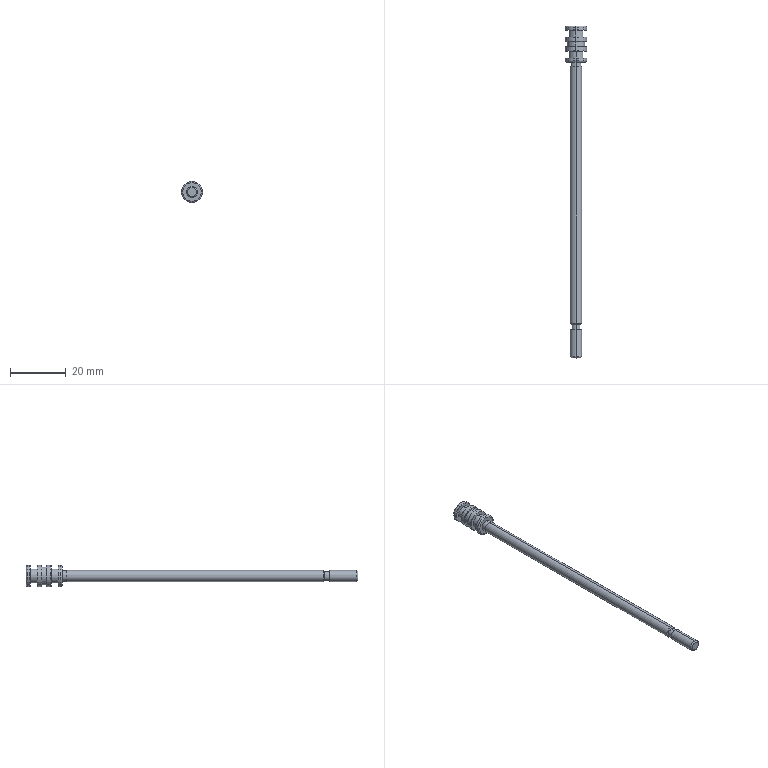Component | SolidWorks | MI-8x60-S-U-M-2(0)-1_MI 8x60-S-U_r-1 | 1 solid | 53 faces | box 7.6 x 119 x 7.6 mm | volume 1755 mm3 | cylinder 22 | cone 16 | plane 11 | torus 4 | commonest cylinder face diameters 7.6 x8 5 x4 4 x4 6.3 x2 3.9 x2 3.2 x2
build123d program:
from build123d import *


with BuildPart() as part:
    # Sketch1 → Revolve1 (revolve)
    with BuildSketch(Plane.XY, mode=Mode.PRIVATE) as revolve1_sk:
        with BuildLine():
            Line((-28, 0), (-28, 1.571))
            Line((-28, 1.571), (-27.57, 2))
            Line((-27.57, 2), (-17.8, 2))
            Line((-17.8, 2), (-17.8, 1.6))
            Line((-17.8, 1.6), (-16, 1.6))
            Line((-16, 1.6), (-15.6, 2))
            Line((-15.6, 2), (76.5, 2))
            Line((76.5, 2), (76.5, 1.95))
            Line((76.5, 1.95), (78, 1.95))
            Line((78, 1.95), (78, 3.3))
            ThreePointArc((78, 3.3), (78.146, 3.654), (78.5, 3.8))
            Line((78.5, 3.8), (79.4, 3.8))
            Line((79.4, 3.8), (79.5, 3.7))
            Line((79.5, 3.7), (79.5, 2.5))
            Line((79.5, 2.5), (82, 2.5))
            Line((82, 2.5), (82, 3.7))
            Line((82, 3.7), (82.1, 3.8))
            Line((82.1, 3.8), (83.55, 3.8))
            Line((83.55, 3.8), (83.65, 3.7))
            Line((83.65, 3.7), (83.65, 3.15))
            Line((83.65, 3.15), (85.35, 3.15))
            Line((85.35, 3.15), (85.35, 3.7))
            Line((85.35, 3.7), (85.45, 3.8))
            Line((85.45, 3.8), (86.9, 3.8))
            Line((86.9, 3.8), (87, 3.7))
            Line((87, 3.7), (87, 2.5))
            Line((87, 2.5), (89.5, 2.5))
            Line((89.5, 2.5), (89.5, 3.7))
            Line((89.5, 3.7), (89.6, 3.8))
            Line((89.6, 3.8), (90.5, 3.8))
            ThreePointArc((90.5, 3.8), (90.854, 3.654), (91, 3.3))
            Line((91, 3.3), (91, 0))
            Line((91, 0), (-28, 0))
        make_face()
    revolve(revolve1_sk.sketch.rotate(Axis((91, 0, 0), (-1, 0, 0)), 270), axis=Axis((91, 0, 0), (-1, 0, 0)))


solid = part.part

# Placed as in the assembly
solid = solid.moved(Location((-44.181, -79.273, -311.979), (0, 0, 90)))